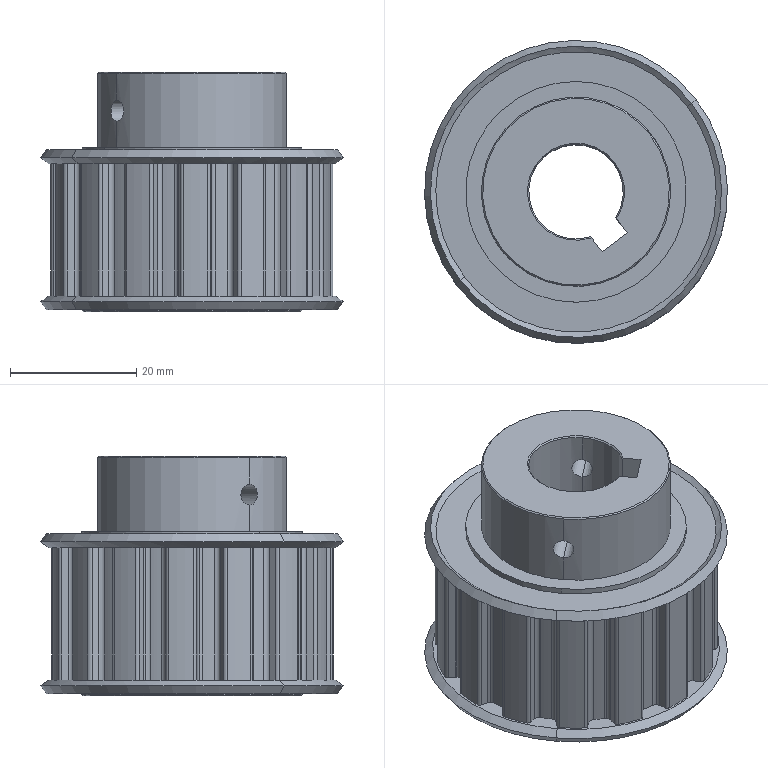Component | SolidWorks | ATPA15L075_B_H15-2-1 | 1 solid | 178 faces | box 48 x 48 x 38 mm | volume 38952 mm3 | cylinder 116 | plane 40 | cone 22 | commonest cylinder face diameters 1.06 x37 1.72 x36 40.46 x15 44.72 x15 3.3 x4 35 x4 15 x3 30 x2
build123d program:
from build123d import *

# Parameters (mm, degrees)
SKETCH2_W          = 89.44
SKETCH2_H          = 89.44
CUT_EXTRUDE1_DEPTH = 21
SKETCH3_W          = 5
SKETCH3_H          = 3
CUT_EXTRUDE2_DEPTH = 51.951
M4_TAPPED_HOLE1_D  = 3.3


with BuildPart() as part:
    # Sketch1 → Revolve1 (revolve)
    with BuildSketch(Plane.XY, mode=Mode.PRIVATE) as revolve1_sk:
        Polygon((0, 17.3), (0, 7.7), (0.2, 7.5), (37.8, 7.5), (38, 7.7), (38, 14.8), (37.8, 15), (26, 15), (26, 17.5), (25.1, 17.5), (25.1, 22.227), (25.702, 23.07), (24.4, 24), (23.5, 22.74), (2.5, 22.74), (1.6, 24), (0.298, 23.07), (0.9, 22.227), (0.9, 17.5), (0.2, 17.5), align=None)
    revolve(revolve1_sk.sketch.rotate(Axis((38, 0, 0), (-1, 0, 0)), 270), axis=Axis((38, 0, 0), (-1, 0, 0)))

    # Sketch2 → Cut-Extrude1 (cut)
    with BuildSketch(Plane(origin=(2.5, 0, 0), x_dir=(0, 0, -1), z_dir=(1, 0, 0))):
        Rectangle(SKETCH2_W, SKETCH2_H)
        with BuildLine():
            Line((-21.955, -0.1348), (-20.845, -0.4115))
            ThreePointArc((-20.845, -0.4115), (-20.391, -0.6967), (-20.195, -1.195))
            ThreePointArc((-20.195, -1.195), (-20.119, -2.115), (-20.002, -3.03))
            ThreePointArc((-20.002, -3.03), (-20.091, -3.558), (-20.475, -3.931))
            Line((-20.475, -3.931), (-21.503, -4.433))
            ThreePointArc((-21.503, -4.433), (-21.749, -4.681), (-21.787, -5.028))
            ThreePointArc((-21.787, -5.028), (-21.547, -5.975), (-21.266, -6.91))
            ThreePointArc((-21.266, -6.91), (-20.944, -7.831), (-20.582, -8.738))
            ThreePointArc((-20.582, -8.738), (-20.347, -8.997), (-20.002, -9.053))
            Line((-20.002, -9.053), (-18.876, -8.854))
            ThreePointArc((-18.876, -8.854), (-18.345, -8.93), (-17.963, -9.306))
            ThreePointArc((-17.963, -9.306), (-17.52, -10.115), (-17.04, -10.903))
            ThreePointArc((-17.04, -10.903), (-16.907, -11.422), (-17.106, -11.92))
            Line((-17.106, -11.92), (-17.841, -12.796))
            ThreePointArc((-17.841, -12.796), (-17.965, -13.122), (-17.858, -13.455))
            ThreePointArc((-17.858, -13.455), (-17.254, -14.222), (-16.617, -14.962))
            ThreePointArc((-16.617, -14.962), (-15.948, -15.673), (-15.248, -16.354))
            ThreePointArc((-15.248, -16.354), (-14.928, -16.495), (-14.591, -16.406))
            Line((-14.591, -16.406), (-13.642, -15.766))
            ThreePointArc((-13.642, -15.766), (-13.127, -15.62), (-12.625, -15.807))
            ThreePointArc((-12.625, -15.807), (-11.891, -16.366), (-11.132, -16.891))
            ThreePointArc((-11.132, -16.891), (-10.799, -17.311), (-10.779, -17.847))
            Line((-10.779, -17.847), (-11.094, -18.946))
            ThreePointArc((-11.094, -18.946), (-11.074, -19.295), (-10.842, -19.556))
            ThreePointArc((-10.842, -19.556), (-9.978, -20.01), (-9.095, -20.427))
            ThreePointArc((-9.095, -20.427), (-8.194, -20.804), (-7.278, -21.142))
            ThreePointArc((-7.278, -21.142), (-6.929, -21.141), (-6.656, -20.922))
            Line((-6.656, -20.922), (-6.05, -19.952))
            ThreePointArc((-6.05, -19.952), (-5.639, -19.609), (-5.104, -19.576))
            ThreePointArc((-5.104, -19.576), (-4.206, -19.788), (-3.3, -19.959))
            ThreePointArc((-3.3, -19.959), (-2.824, -20.207), (-2.588, -20.688))
            Line((-2.588, -20.688), (-2.429, -21.821))
            ThreePointArc((-2.429, -21.821), (-2.269, -22.131), (-1.95, -22.275))
            ThreePointArc((-1.95, -22.275), (-0.9761, -22.339), (0, -22.36))
            ThreePointArc((0, -22.36), (0.9761, -22.339), (1.95, -22.275))
            ThreePointArc((1.95, -22.275), (2.269, -22.131), (2.429, -21.821))
            Line((2.429, -21.821), (2.588, -20.688))
            ThreePointArc((2.588, -20.688), (2.824, -20.207), (3.3, -19.959))
            ThreePointArc((3.3, -19.959), (4.206, -19.788), (5.104, -19.576))
            ThreePointArc((5.104, -19.576), (5.639, -19.609), (6.05, -19.952))
            Line((6.05, -19.952), (6.656, -20.922))
            ThreePointArc((6.656, -20.922), (6.929, -21.141), (7.278, -21.142))
            ThreePointArc((7.278, -21.142), (8.194, -20.804), (9.095, -20.427))
            ThreePointArc((9.095, -20.427), (9.978, -20.01), (10.842, -19.556))
            ThreePointArc((10.842, -19.556), (11.074, -19.295), (11.094, -18.946))
            Line((11.094, -18.946), (10.779, -17.847))
            ThreePointArc((10.779, -17.847), (10.799, -17.311), (11.132, -16.891))
            ThreePointArc((11.132, -16.891), (11.891, -16.366), (12.625, -15.807))
            ThreePointArc((12.625, -15.807), (13.127, -15.62), (13.642, -15.766))
            Line((13.642, -15.766), (14.591, -16.406))
            ThreePointArc((14.591, -16.406), (14.928, -16.495), (15.248, -16.354))
            ThreePointArc((15.248, -16.354), (15.948, -15.673), (16.617, -14.962))
            ThreePointArc((16.617, -14.962), (17.254, -14.222), (17.858, -13.455))
            ThreePointArc((17.858, -13.455), (17.965, -13.122), (17.841, -12.796))
            Line((17.841, -12.796), (17.106, -11.92))
            ThreePointArc((17.106, -11.92), (16.907, -11.422), (17.04, -10.903))
            ThreePointArc((17.04, -10.903), (17.52, -10.115), (17.963, -9.306))
            ThreePointArc((17.963, -9.306), (18.345, -8.93), (18.876, -8.854))
            Line((18.876, -8.854), (20.002, -9.053))
            ThreePointArc((20.002, -9.053), (20.347, -8.997), (20.582, -8.738))
            ThreePointArc((20.582, -8.738), (20.944, -7.831), (21.266, -6.91))
            ThreePointArc((21.266, -6.91), (21.547, -5.975), (21.787, -5.028))
            ThreePointArc((21.787, -5.028), (21.749, -4.681), (21.503, -4.433))
            Line((21.503, -4.433), (20.475, -3.931))
            ThreePointArc((20.475, -3.931), (20.091, -3.558), (20.002, -3.03))
            ThreePointArc((20.002, -3.03), (20.119, -2.115), (20.195, -1.195))
            ThreePointArc((20.195, -1.195), (20.391, -0.6967), (20.845, -0.4115))
            Line((20.845, -0.4115), (21.955, -0.1348))
            ThreePointArc((21.955, -0.1348), (22.247, 0.05676), (22.357, 0.3886))
            ThreePointArc((22.357, 0.3886), (22.318, 1.364), (22.238, 2.337))
            ThreePointArc((22.238, 2.337), (22.114, 3.306), (21.949, 4.268))
            ThreePointArc((21.949, 4.268), (21.773, 4.57), (21.447, 4.697))
            Line((21.447, 4.697), (20.304, 4.736))
            ThreePointArc((20.304, 4.736), (19.801, 4.921), (19.505, 5.368))
            ThreePointArc((19.505, 5.368), (19.24, 6.251), (18.935, 7.122))
            ThreePointArc((18.935, 7.122), (18.912, 7.657), (19.21, 8.103))
            Line((19.21, 8.103), (20.112, 8.807))
            ThreePointArc((20.112, 8.807), (20.301, 9.101), (20.266, 9.448))
            ThreePointArc((20.266, 9.448), (19.834, 10.324), (19.364, 11.18))
            ThreePointArc((19.364, 11.18), (18.858, 12.015), (18.315, 12.826))
            ThreePointArc((18.315, 12.826), (18.032, 13.031), (17.683, 13.014))
            Line((17.683, 13.014), (16.622, 12.585))
            ThreePointArc((16.622, 12.585), (16.087, 12.549), (15.635, 12.837))
            ThreePointArc((15.635, 12.837), (15.034, 13.537), (14.401, 14.208))
            ThreePointArc((14.401, 14.208), (14.162, 14.688), (14.254, 15.216))
            Line((14.254, 15.216), (14.791, 16.225))
            ThreePointArc((14.791, 16.225), (14.844, 16.571), (14.671, 16.874))
            ThreePointArc((14.671, 16.874), (13.92, 17.499), (13.143, 18.09))
            ThreePointArc((13.143, 18.09), (12.341, 18.646), (11.515, 19.167))
            ThreePointArc((11.515, 19.167), (11.173, 19.238), (10.861, 19.081))
            Line((10.861, 19.081), (10.066, 18.258))
            ThreePointArc((10.066, 18.258), (9.592, 18.008), (9.062, 18.087))
            ThreePointArc((9.062, 18.087), (8.228, 18.481), (7.377, 18.837))
            ThreePointArc((7.377, 18.837), (6.964, 19.178), (6.833, 19.698))
            Line((6.833, 19.698), (6.913, 20.839))
            ThreePointArc((6.913, 20.839), (6.821, 21.176), (6.539, 21.383))
            ThreePointArc((6.539, 21.383), (5.599, 21.648), (4.649, 21.871))
            ThreePointArc((4.649, 21.871), (3.69, 22.053), (2.723, 22.194))
            ThreePointArc((2.723, 22.194), (2.382, 22.119), (2.161, 21.849))
            Line((2.161, 21.849), (1.77, 20.774))
            ThreePointArc((1.77, 20.774), (1.439, 20.353), (0.9223, 20.209))
            ThreePointArc((0.9223, 20.209), (0, 20.23), (-0.9223, 20.209))
            ThreePointArc((-0.9223, 20.209), (-1.439, 20.353), (-1.77, 20.774))
            Line((-1.77, 20.774), (-2.161, 21.849))
            ThreePointArc((-2.161, 21.849), (-2.382, 22.119), (-2.723, 22.194))
            ThreePointArc((-2.723, 22.194), (-3.69, 22.053), (-4.649, 21.871))
            ThreePointArc((-4.649, 21.871), (-5.599, 21.648), (-6.539, 21.383))
            ThreePointArc((-6.539, 21.383), (-6.821, 21.176), (-6.913, 20.839))
            Line((-6.913, 20.839), (-6.833, 19.698))
            ThreePointArc((-6.833, 19.698), (-6.964, 19.178), (-7.377, 18.837))
            ThreePointArc((-7.377, 18.837), (-8.228, 18.481), (-9.062, 18.087))
            ThreePointArc((-9.062, 18.087), (-9.592, 18.008), (-10.066, 18.258))
            Line((-10.066, 18.258), (-10.861, 19.081))
            ThreePointArc((-10.861, 19.081), (-11.173, 19.238), (-11.515, 19.167))
            ThreePointArc((-11.515, 19.167), (-12.341, 18.646), (-13.143, 18.09))
            ThreePointArc((-13.143, 18.09), (-13.92, 17.499), (-14.671, 16.874))
            ThreePointArc((-14.671, 16.874), (-14.844, 16.571), (-14.791, 16.225))
            Line((-14.791, 16.225), (-14.254, 15.216))
            ThreePointArc((-14.254, 15.216), (-14.162, 14.688), (-14.401, 14.208))
            ThreePointArc((-14.401, 14.208), (-15.034, 13.537), (-15.635, 12.837))
            ThreePointArc((-15.635, 12.837), (-16.087, 12.549), (-16.622, 12.585))
            Line((-16.622, 12.585), (-17.683, 13.014))
            ThreePointArc((-17.683, 13.014), (-18.032, 13.031), (-18.315, 12.826))
            ThreePointArc((-18.315, 12.826), (-18.858, 12.015), (-19.364, 11.18))
            ThreePointArc((-19.364, 11.18), (-19.834, 10.324), (-20.266, 9.448))
            ThreePointArc((-20.266, 9.448), (-20.301, 9.101), (-20.112, 8.807))
            Line((-20.112, 8.807), (-19.21, 8.103))
            ThreePointArc((-19.21, 8.103), (-18.912, 7.657), (-18.935, 7.122))
            ThreePointArc((-18.935, 7.122), (-19.24, 6.251), (-19.505, 5.368))
            ThreePointArc((-19.505, 5.368), (-19.801, 4.921), (-20.304, 4.736))
            Line((-20.304, 4.736), (-21.447, 4.697))
            ThreePointArc((-21.447, 4.697), (-21.773, 4.57), (-21.949, 4.268))
            ThreePointArc((-21.949, 4.268), (-22.114, 3.306), (-22.238, 2.337))
            ThreePointArc((-22.238, 2.337), (-22.318, 1.364), (-22.357, 0.3886))
            ThreePointArc((-22.357, 0.3886), (-22.247, 0.05676), (-21.955, -0.1348))
        make_face(mode=Mode.SUBTRACT)
    extrude(amount=CUT_EXTRUDE1_DEPTH, mode=Mode.SUBTRACT)

    # Sketch3 → Cut-Extrude2 (cut, through all)
    with BuildSketch(Plane(origin=(38, 0, 0), x_dir=(0, 0, -1), z_dir=(1, 0, 0))):
        with Locations((0, 8.571)):
            Rectangle(SKETCH3_W, SKETCH3_H)
    extrude(amount=-CUT_EXTRUDE2_DEPTH, mode=Mode.SUBTRACT)

    # M4 Tapped Hole1 (through all)
    with Locations(Plane(origin=(0, 0, -15), x_dir=(1, 0, 0), z_dir=(0, 0, -1))):
        with Locations((31.9, 0)):
            Hole(M4_TAPPED_HOLE1_D / 2)


solid = part.part

# Placed as in the assembly
solid = solid.moved(Location((647.283, -168.115, -199), (-90, 52.559, -89.999)))